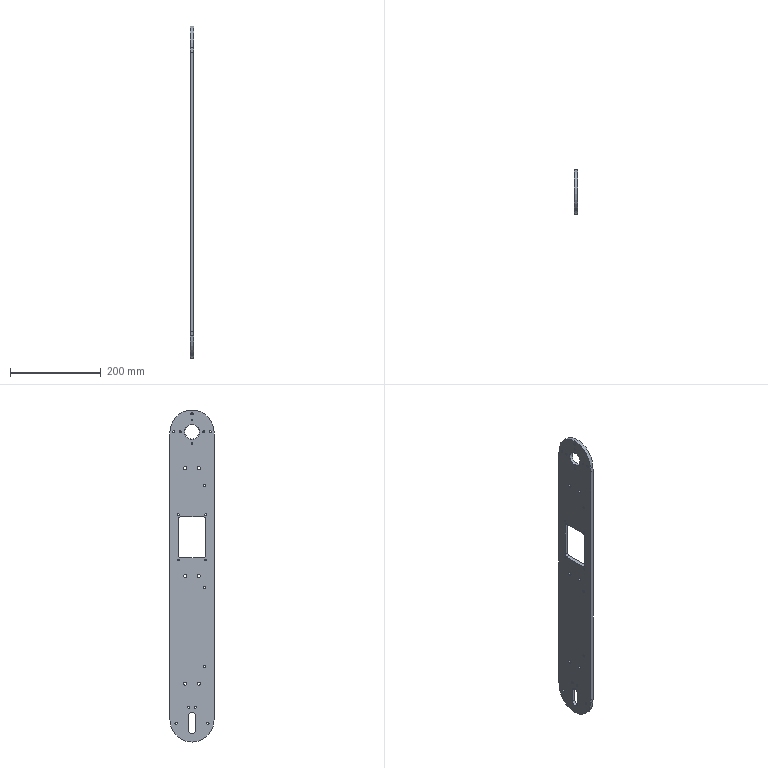Component | SolidWorks | ChainPartOuterSidePlate-1 | 1 solid | 78 faces | box 8 x 99 x 732 mm | volume 502720 mm3 | cylinder 60 | plane 14 | cone 4 | commonest cylinder face diameters 5 x20 4 x16 7 x12 10 x4 97 x3 16 x3 32 x2
build123d program:
from build123d import *

# Parameters (mm, degrees)
BOSS_EXTRUDE1_DEPTH = 4
SKETCH3_R           = 16
CUT_EXTRUDE2_DEPTH  = 371.41
CUT_EXTRUDE3_DEPTH  = 10
M4_TAPPED_HOLE1_D   = 4
CHAMFER1_SIZE       = 0.5
SKETCH7_R           = 3.5
CUT_EXTRUDE4_DEPTH  = 10
CUT_EXTRUDE5_DEPTH  = 371.41
M4_TAPPED_HOLE2_D   = 4
M5_TAPPED_HOLE1_D   = 5
CUT_EXTRUDE6_DEPTH  = 371.41
M5_TAPPED_HOLE2_D   = 5
M5_TAPPED_HOLE3_D   = 5
M5_TAPPED_HOLE4_D   = 5


with BuildPart() as part:
    # Sketch1 → Boss-Extrude1 (new, symmetric)
    with BuildSketch(Plane.XY):
        with BuildLine():
            Line((-317.5, 49.5), (317.5, 49.5))
            ThreePointArc((317.5, 49.5), (367, 0), (317.5, -49.5))
            Line((317.5, -49.5), (-317.5, -49.5))
            ThreePointArc((-317.5, -49.5), (-367, 0), (-317.5, 49.5))
        make_face()
    extrude(amount=BOSS_EXTRUDE1_DEPTH, both=True)

    # Sketch3 → Cut-Extrude2 (cut, through all)
    with BuildSketch(Plane.XY.offset(4)):
        with Locations((-317.5, 0)):
            Circle(SKETCH3_R)
    extrude(amount=-CUT_EXTRUDE2_DEPTH, mode=Mode.SUBTRACT)

    # Sketch4 → Cut-Extrude3 (cut)
    with BuildSketch(Plane.XY.offset(4)):
        with BuildLine():
            Line((309.5, 8), (339.5, 8))
            ThreePointArc((339.5, 8), (347.5, 0), (339.5, -8))
            Line((339.5, -8), (309.5, -8))
            ThreePointArc((309.5, -8), (301.5, 0), (309.5, 8))
        make_face()
    extrude(amount=-CUT_EXTRUDE3_DEPTH, mode=Mode.SUBTRACT)

    # M4 Tapped Hole1 (through all)
    with Locations(Plane(origin=(0, 0, -4), x_dir=(-1, 0, 0), z_dir=(0, 0, -1))):
        with Locations((317.5, 26), (291.5, 0), (317.5, -26), (343.5, 0)):
            Hole(M4_TAPPED_HOLE1_D / 2)

    # Chamfer1
    chamfer1_edges = [part.edges().sort_by_distance(p)[0] for p in [
        (-333.5, 0, -4),
        (-333.5, 0, 4),
    ]]
    chamfer(chamfer1_edges, length=CHAMFER1_SIZE)

    # Sketch7 → Cut-Extrude4 (cut)
    with BuildSketch(Plane(origin=(0, 0, -4), x_dir=(-1, 0, 0), z_dir=(0, 0, -1))):
        with Locations((237.5, 15)):
            Circle(SKETCH7_R)
        with Locations((237.5, -15)):
            Circle(SKETCH7_R)
        with Locations((-237.5, 15)):
            Circle(SKETCH7_R)
        with Locations((-237.5, -15)):
            Circle(SKETCH7_R)
        with Locations((0, 15)):
            Circle(SKETCH7_R)
        with Locations((0, -15)):
            Circle(SKETCH7_R)
    extrude(amount=-CUT_EXTRUDE4_DEPTH, mode=Mode.SUBTRACT)

    # Sketch8 → Cut-Extrude5 (cut, through all)
    with BuildSketch(Plane.XY.offset(4)):
        with BuildLine():
            Line((-125, 30), (-45, 30))
            ThreePointArc((-45, 30), (-41.464, 28.536), (-40, 25))
            Line((-40, 25), (-40, -25))
            ThreePointArc((-40, -25), (-41.464, -28.536), (-45, -30))
            Line((-45, -30), (-125, -30))
            ThreePointArc((-125, -30), (-128.536, -28.536), (-130, -25))
            Line((-130, -25), (-130, 25))
            ThreePointArc((-130, 25), (-128.536, 28.536), (-125, 30))
        make_face()
    extrude(amount=-CUT_EXTRUDE5_DEPTH, mode=Mode.SUBTRACT)

    # M4 Tapped Hole2 (through all)
    with Locations(Plane.XY.offset(4)):
        with Locations((-135, 30), (-135, -30), (-35, 30), (-35, -30)):
            Hole(M4_TAPPED_HOLE2_D / 2)

    # M5 Tapped Hole1 (through all)
    with Locations(Plane.XY.offset(4)):
        with Locations((-317.5, 40), (-357.5, 0), (-317.5, -40)):
            Hole(M5_TAPPED_HOLE1_D / 2)

    # Sketch13 → Cut-Extrude6 (cut, through all)
    with BuildSketch(Plane.XY.offset(4)):
        with BuildLine():
            Line((-307.5, 49.5), (-317.5, 48.5))
            ThreePointArc((-317.5, 48.5), (-366, 0), (-317.5, -48.5))
            Line((-317.5, -48.5), (-307.5, -49.5))
            Line((-307.5, -49.5), (-317.5, -49.5))
            ThreePointArc((-317.5, -49.5), (-367, 0), (-317.5, 49.5))
            Line((-317.5, 49.5), (-307.5, 49.5))
        make_face()
        with BuildLine():
            Line((307.5, 49.5), (317.5, 48.5))
            ThreePointArc((317.5, 48.5), (366, 0), (317.5, -48.5))
            Line((317.5, -48.5), (307.5, -49.5))
            Line((307.5, -49.5), (317.5, -49.5))
            ThreePointArc((317.5, -49.5), (367, 0), (317.5, 49.5))
            Line((317.5, 49.5), (307.5, 49.5))
        make_face()
    extrude(amount=-CUT_EXTRUDE6_DEPTH, mode=Mode.SUBTRACT)

    # M5 Tapped Hole2 (through all)
    with Locations(Plane.XY.offset(4)):
        with Locations((289.5, 7), (289.5, -7)):
            Hole(M5_TAPPED_HOLE2_D / 2)

    # M5 Tapped Hole3 (through all)
    with Locations(Plane.XY.offset(4)):
        with Locations((324.5, 35), (324.5, -35)):
            Hole(M5_TAPPED_HOLE3_D / 2)

    # M5 Tapped Hole4 (through all)
    with Locations(Plane.XY.offset(4)):
        with Locations((-200, 28), (200, 28), (25, 28)):
            Hole(M5_TAPPED_HOLE4_D / 2)


solid = part.part

# Placed as in the assembly
solid = solid.moved(Location((84.237, -2.563, -352.804), (180, -90, 0)))